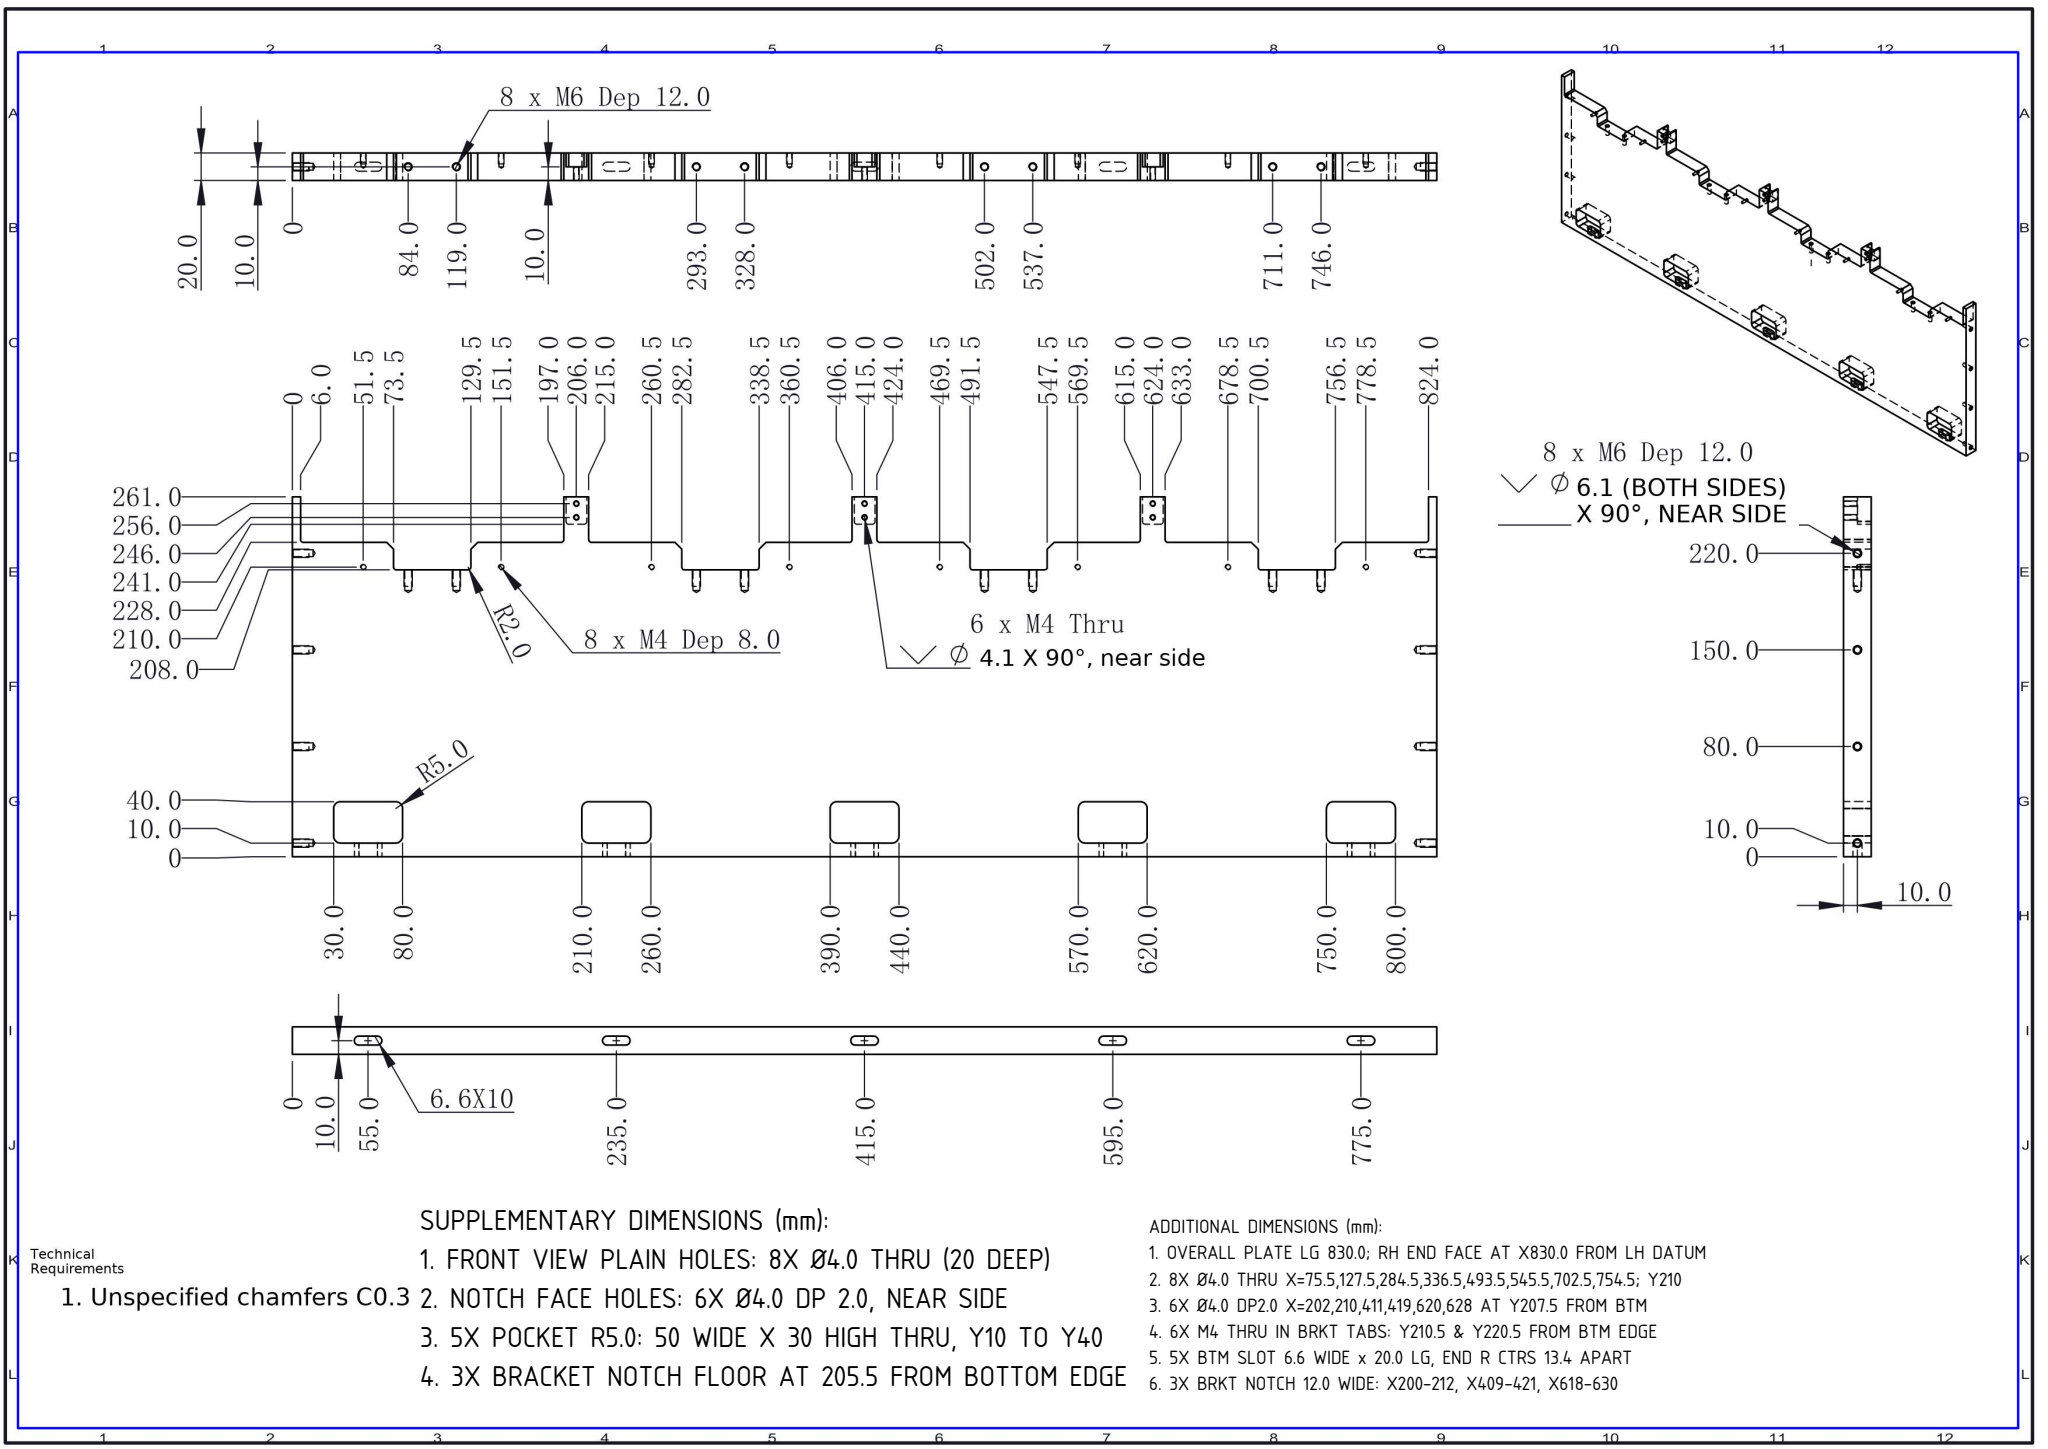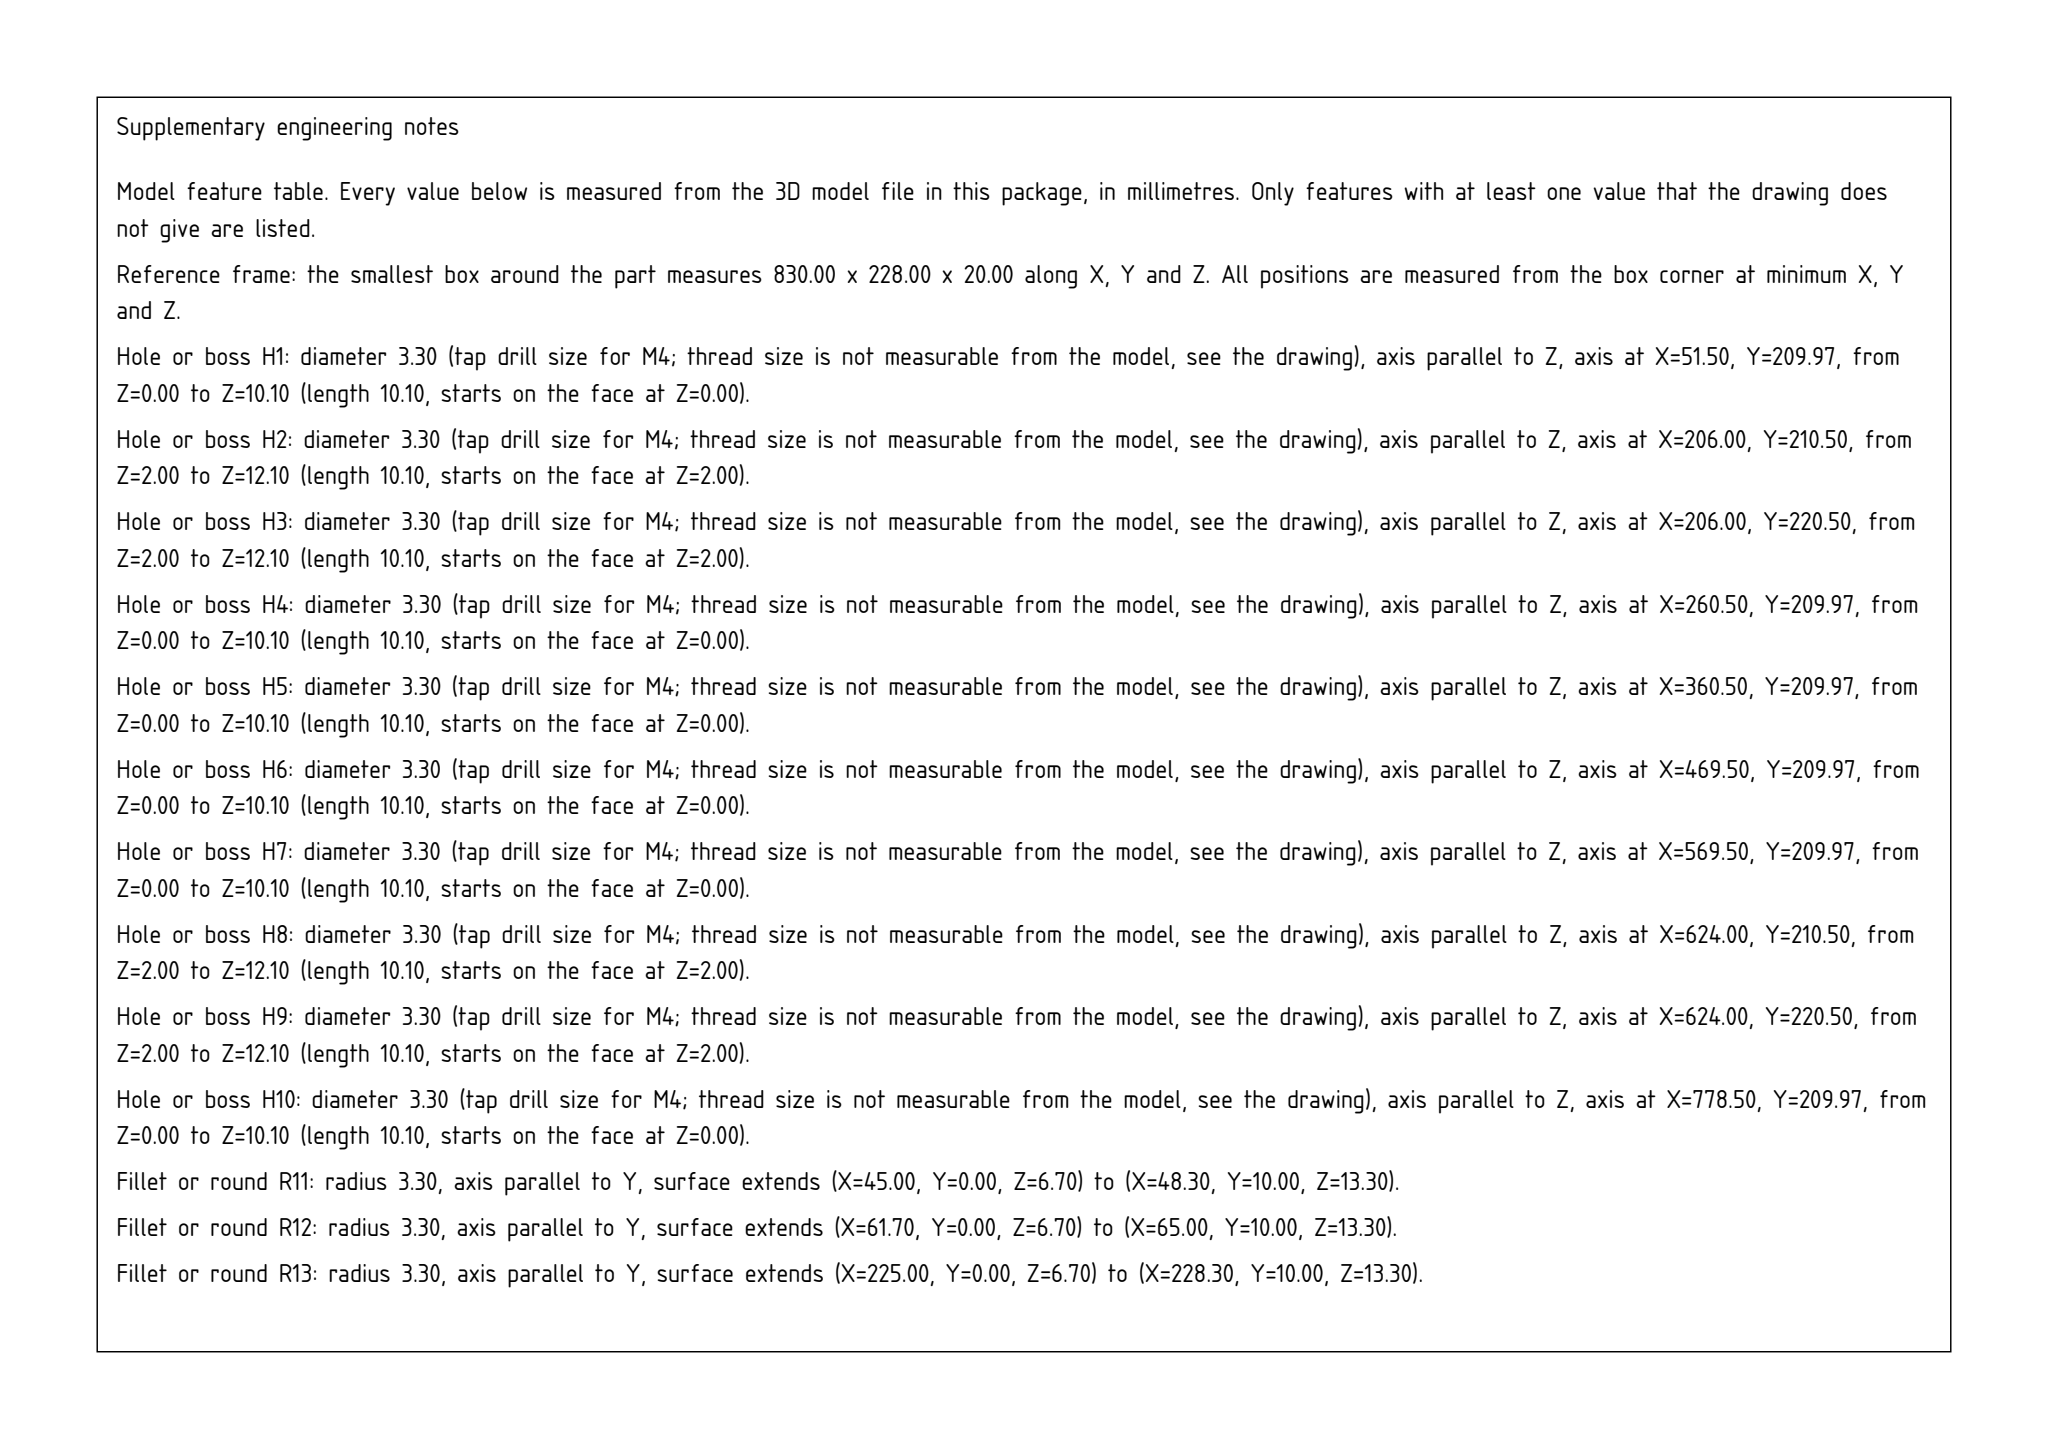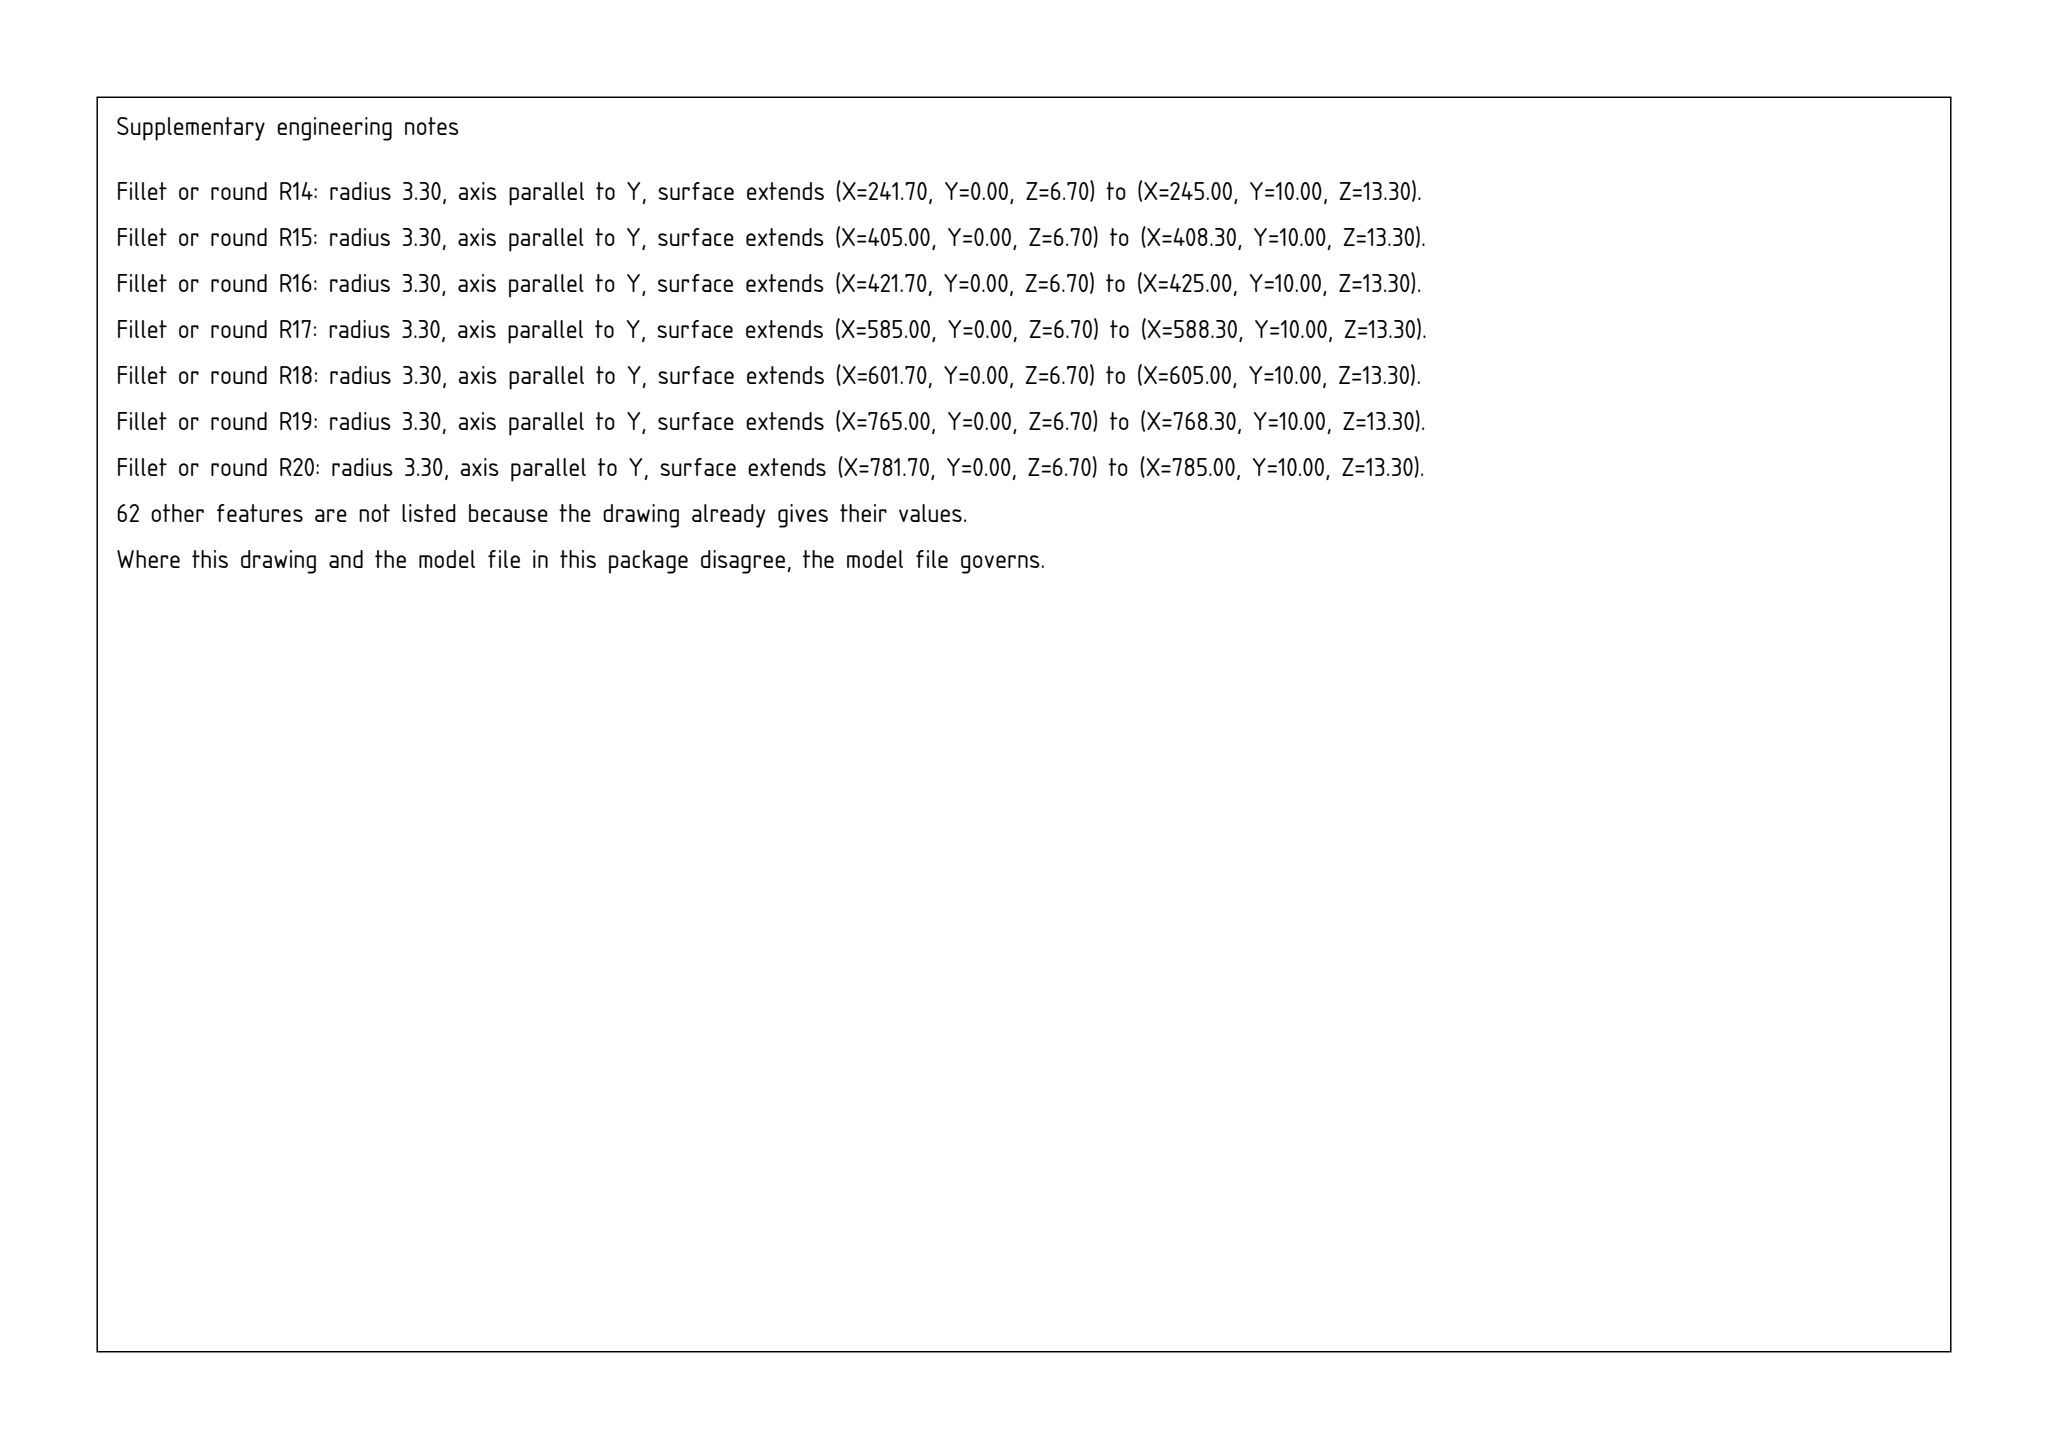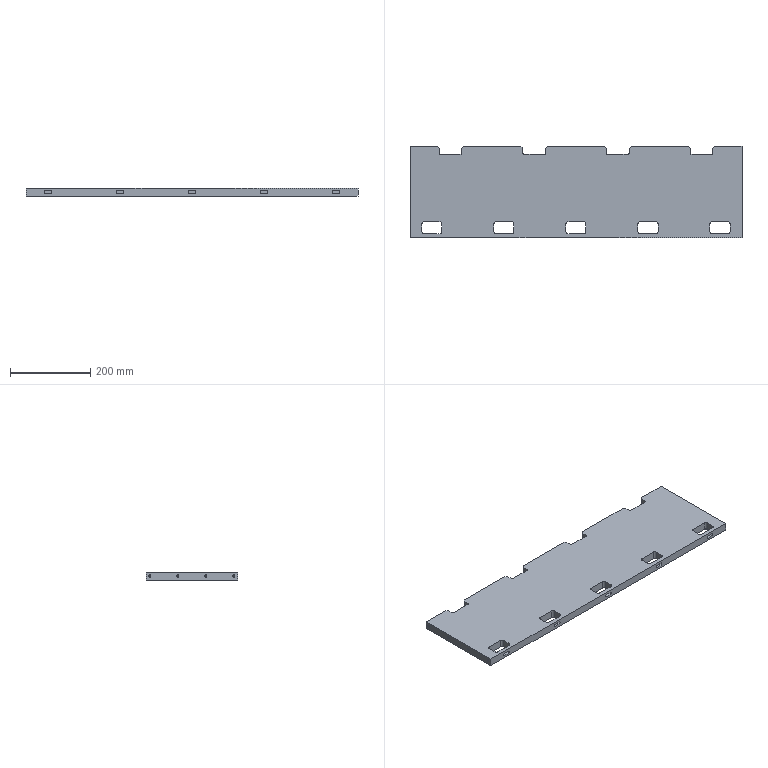Part | SolidWorks | mm | 1 solid | 252 faces | box 830 x 228 x 20 mm | volume 3531604 mm3 | cylinder 104 | cone 76 | plane 72 | commonest cylinder face diameters 5 x32 3.3 x28 10 x20 4 x14 6.6 x10